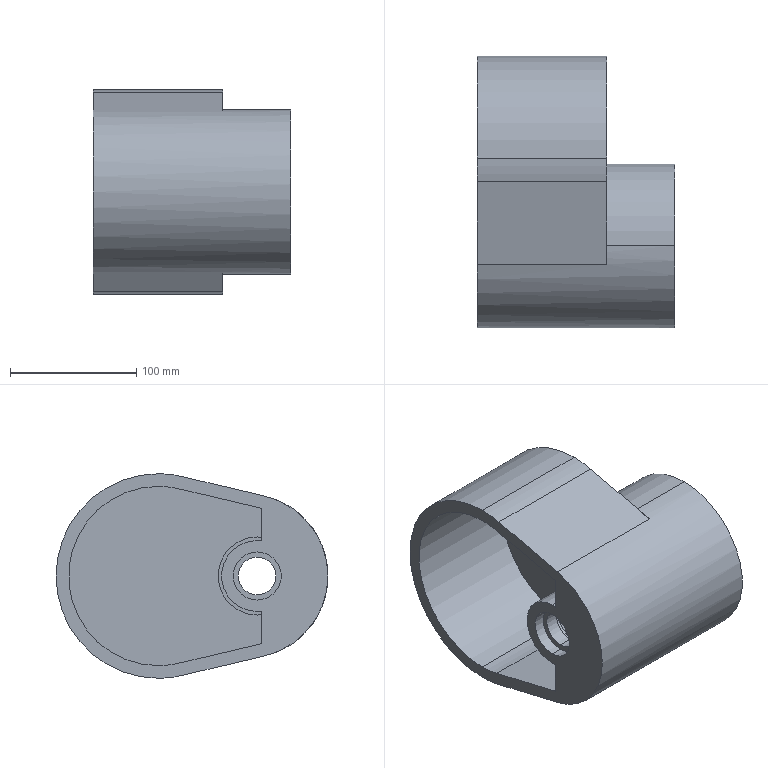Component | SolidWorks | Gearbox-1 | 1 solid | 42 faces | box 157 x 215.66 x 162.15 mm | volume 1446902 mm3 | cylinder 25 | plane 17 | commonest cylinder face diameters 142.145 x3 162.145 x3 7 x2 46.464 x2 38.185 x2 56.248 x2 61.875 x2 51.14 x2
build123d program:
from build123d import *

# Parameters (mm, degrees)
SKETCH2_R           = 65.149
BOSS_EXTRUDE1_DEPTH = 54
BOSS_EXTRUDE2_DEPTH = 103
SKETCH4_R           = 18.564
CUT_EXTRUDE1_DEPTH  = 15
SKETCH5_R           = 25.57
CUT_EXTRUDE2_DEPTH  = 10
CUT_EXTRUDE3_DEPTH  = 93
SKETCH7_R           = 30.938
CUT_EXTRUDE5_DEPTH  = 10
SKETCH10_R          = 25.57
CUT_EXTRUDE7_DEPTH  = 109
SKETCH11_R          = 28.124
BOSS_EXTRUDE3_DEPTH = 28
SKETCH12_R          = 28.124
BOSS_EXTRUDE4_DEPTH = 5
SKETCH13_R          = 19.092
CUT_EXTRUDE9_DEPTH  = 9
SKETCH14_R          = 15
CUT_EXTRUDE10_DEPTH = 19
CUT_EXTRUDE11_START = -8
SKETCH15_R          = 23.232
SKETCH15_R_2        = 15
CUT_EXTRUDE11_DEPTH = 8
SKETCH16_R          = 3.5
CUT_EXTRUDE13_DEPTH = 29


with BuildPart() as part:
    # Sketch2 → Boss-Extrude1 (new body)
    with BuildSketch(Plane.XY):
        with Locations((0, 69.2)):
            Circle(SKETCH2_R)
    extrude(amount=BOSS_EXTRUDE1_DEPTH)

    # Sketch3 → Boss-Extrude2 (add)
    with BuildSketch(Plane.XY.offset(54)):
        with BuildLine():
            Line((78.912, 120.041), (63.412, 54.259))
            ThreePointArc((63.412, 54.259), (0, 4.051), (-63.412, 54.259))
            Line((-63.412, 54.259), (-78.912, 120.041))
            ThreePointArc((-78.912, 120.041), (0, 219.707), (78.912, 120.041))
        make_face()
    extrude(amount=BOSS_EXTRUDE2_DEPTH)

    # Sketch4 → Cut-Extrude1 (cut)
    with BuildSketch(Plane(origin=(0, 0, 0), x_dir=(-1, 0, 0), z_dir=(0, 0, -1))):
        with Locations((0, 60.219)):
            Circle(SKETCH4_R)
    extrude(amount=-CUT_EXTRUDE1_DEPTH, mode=Mode.SUBTRACT)

    # Sketch5 → Cut-Extrude2 (cut)
    with BuildSketch(Plane(origin=(0, 0, 15), x_dir=(-1, 0, 0), z_dir=(0, 0, -1))):
        with Locations((0, 60.219)):
            Circle(SKETCH5_R)
    extrude(amount=-CUT_EXTRUDE2_DEPTH, mode=Mode.SUBTRACT)

    # Sketch6 → Cut-Extrude3 (cut)
    with BuildSketch(Plane.XY.offset(157)):
        with BuildLine():
            Line((-69.178, 122.335), (-53.679, 56.552))
            ThreePointArc((-53.679, 56.552), (0, 14.051), (53.679, 56.552))
            Line((53.679, 56.552), (69.178, 122.335))
            ThreePointArc((69.178, 122.335), (0, 209.707), (-69.178, 122.335))
        make_face()
    extrude(amount=-CUT_EXTRUDE3_DEPTH, mode=Mode.SUBTRACT)

    # Sketch7 → Cut-Extrude5 (cut)
    with BuildSketch(Plane.XY.offset(64)):
        with Locations((0, 60.219)):
            Circle(SKETCH7_R)
    extrude(amount=-CUT_EXTRUDE5_DEPTH, mode=Mode.SUBTRACT)

    # Sketch10 → Cut-Extrude7 (cut)
    with BuildSketch(Plane(origin=(0, 0, 25), x_dir=(-1, 0, 0), z_dir=(0, 0, -1))):
        with Locations((0, 60.219)):
            Circle(SKETCH10_R)
    extrude(amount=-CUT_EXTRUDE7_DEPTH, mode=Mode.SUBTRACT)



with BuildPart() as body_2:
    # Sketch11 → Boss-Extrude3 (new body)
    with BuildSketch(Plane.XY.offset(157)):
        with Locations((0, 60.219)):
            Circle(SKETCH11_R)
    extrude(amount=-BOSS_EXTRUDE3_DEPTH)


with BuildPart() as part_1:
    add(part.part)

    add(body_2.part)  # Boss-Extrude4 merges body 2
    # Sketch12 → Boss-Extrude4 (add)
    with BuildSketch(Plane.XY.offset(157)):
        with Locations((0, 60.219)):
            Circle(SKETCH12_R)
        with BuildLine():
            Line((-53.679, 56.552), (53.679, 56.552))
            ThreePointArc((53.679, 56.552), (0, 14.051), (-53.679, 56.552))
        make_face()
    extrude(amount=-BOSS_EXTRUDE4_DEPTH)

    # Sketch13 → Cut-Extrude9 (cut)
    with BuildSketch(Plane.XY.offset(157)):
        with Locations((0, 60.219)):
            Circle(SKETCH13_R)
    extrude(amount=-CUT_EXTRUDE9_DEPTH, mode=Mode.SUBTRACT)

    # Sketch14 → Cut-Extrude10 (cut)
    with BuildSketch(Plane.XY.offset(148)):
        with Locations((0, 60.219)):
            Circle(SKETCH14_R)
    extrude(amount=-CUT_EXTRUDE10_DEPTH, mode=Mode.SUBTRACT)

    # Sketch15 → Cut-Extrude11 (cut)
    with BuildSketch(Plane(origin=(0, 0, 129), x_dir=(-1, 0, 0), z_dir=(0, 0, -1)).offset(CUT_EXTRUDE11_START)):
        with Locations((0, 60.219)):
            Circle(SKETCH15_R)
        with Locations(Location((0, 60.219, 0), (0, 0, 180))):
            Circle(SKETCH15_R_2, mode=Mode.SUBTRACT)
    extrude(amount=CUT_EXTRUDE11_DEPTH, mode=Mode.SUBTRACT)

    # Sketch16 → Cut-Extrude13 (cut)
    with BuildSketch(Plane(origin=(0, 0, 0), x_dir=(-1, 0, 0), z_dir=(0, 0, -1))):
        with Locations((0, 12.224)):
            Circle(SKETCH16_R)
    extrude(amount=-CUT_EXTRUDE13_DEPTH, mode=Mode.SUBTRACT)


solid = part_1.part

# Placed as in the assembly
solid = solid.moved(Location((-277, 0, 0), (0, -90, 0)))